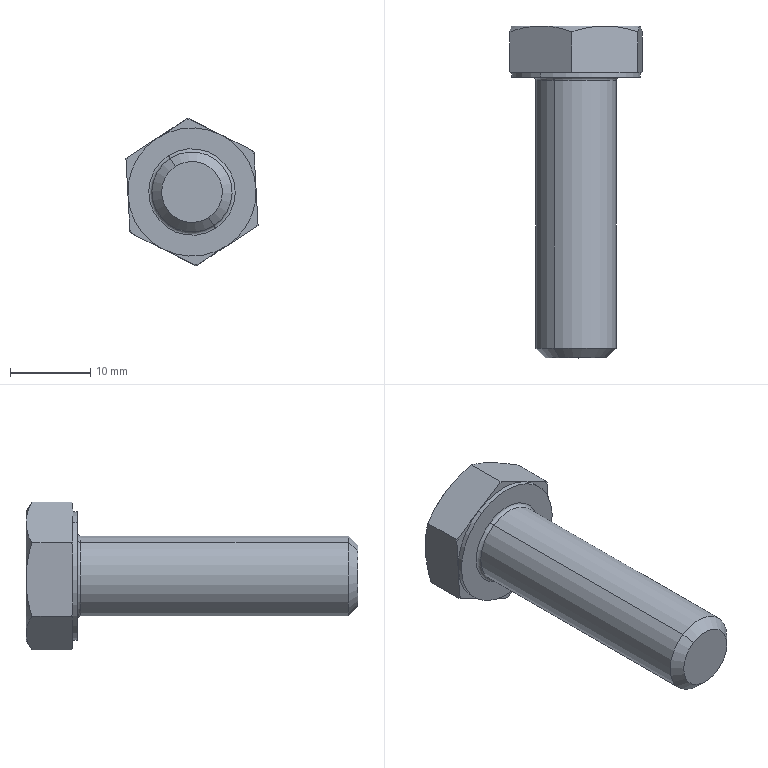Component | SolidWorks | 14HexHeadBolt_GradeAAndB[GBT5782-2000][M10_35_35]-1 | 1 solid | 35 faces | box 16.48 x 41.4 x 18.45 mm | volume 4131 mm3 | plane 15 | cone 14 | cylinder 4 | torus 2 | commonest cylinder face diameters 10 x2 16 x2 | material Steel
STEP:
#1=COLOUR_RGB('',0.7922,0.8196,0.9333);
#2=FILL_AREA_STYLE_COLOUR('',#1);
#3=FILL_AREA_STYLE('',(#2));
#4=SURFACE_STYLE_FILL_AREA(#3);
#5=SURFACE_SIDE_STYLE('',(#4));
#6=SURFACE_STYLE_USAGE(.BOTH.,#5);
#7=PRESENTATION_STYLE_ASSIGNMENT((#6));
#8=CARTESIAN_POINT('',(-7.986,6.04,16.976));
#9=VERTEX_POINT('',#8);
#10=CARTESIAN_POINT('',(-7.771,6.04,16.646));
#11=VERTEX_POINT('',#10);
#12=CARTESIAN_POINT('',(-7.879,6.04,16.811));
#13=DIRECTION('',(0.,-1.,0.));
#14=DIRECTION('',(0.5469,0.,-0.8372));
#15=AXIS2_PLACEMENT_3D('',#12,#13,#14);
#16=CIRCLE('',#15,0.1969);
#17=EDGE_CURVE('',#9,#11,#16,.T.);
#18=ORIENTED_EDGE('',*,*,#17,.F.);
#19=CARTESIAN_POINT('',(-7.995,6.055,16.989));
#20=VERTEX_POINT('',#19);
#21=CARTESIAN_POINT('',(-7.995,6.04,16.989));
#22=DIRECTION('',(0.8372,0.,0.5469));
#23=DIRECTION('',(0.5469,0.,-0.8372));
#24=AXIS2_PLACEMENT_3D('',#21,#22,#23);
#25=CIRCLE('',#24,0.01575);
#26=EDGE_CURVE('',#9,#20,#25,.T.);
#27=ORIENTED_EDGE('',*,*,#26,.T.);
#28=CARTESIAN_POINT('',(-7.762,6.055,16.633));
#29=VERTEX_POINT('',#28);
#30=CARTESIAN_POINT('',(-7.879,6.055,16.811));
#31=DIRECTION('',(0.,1.,0.));
#32=DIRECTION('',(0.5469,0.,-0.8372));
#33=AXIS2_PLACEMENT_3D('',#30,#31,#32);
#34=CIRCLE('',#33,0.2126);
#35=EDGE_CURVE('',#29,#20,#34,.T.);
#36=ORIENTED_EDGE('',*,*,#35,.F.);
#37=CARTESIAN_POINT('',(-7.762,6.04,16.633));
#38=DIRECTION('',(-0.8372,0.,-0.5469));
#39=DIRECTION('',(-0.5469,0.,0.8372));
#40=AXIS2_PLACEMENT_3D('',#37,#38,#39);
#41=CIRCLE('',#40,0.01575);
#42=EDGE_CURVE('',#11,#29,#41,.T.);
#43=ORIENTED_EDGE('',*,*,#42,.F.);
#44=EDGE_LOOP('',(#18,#27,#36,#43));
#45=FACE_OUTER_BOUND('',#44,.T.);
#46=CARTESIAN_POINT('',(-7.879,6.04,16.811));
#47=DIRECTION('',(0.,-1.,0.));
#48=DIRECTION('',(0.5469,0.,-0.8372));
#49=AXIS2_PLACEMENT_3D('',#46,#47,#48);
#50=TOROIDAL_SURFACE('',#49,0.2126,0.01575);
#51=ADVANCED_FACE('',(#45),#50,.F.);
#52=CARTESIAN_POINT('',(-7.797,4.678,16.686));
#53=VERTEX_POINT('',#52);
#54=CARTESIAN_POINT('',(-7.96,4.678,16.936));
#55=VERTEX_POINT('',#54);
#56=CARTESIAN_POINT('',(-7.879,4.678,16.811));
#57=DIRECTION('',(0.,-1.,0.));
#58=DIRECTION('',(-0.5469,0.,0.8372));
#59=AXIS2_PLACEMENT_3D('',#56,#57,#58);
#60=CIRCLE('',#59,0.1496);
#61=EDGE_CURVE('',#53,#55,#60,.T.);
#62=ORIENTED_EDGE('',*,*,#61,.F.);
#63=CARTESIAN_POINT('',(-7.771,4.725,16.646));
#64=VERTEX_POINT('',#63);
#65=CARTESIAN_POINT('',(-7.771,4.725,16.646));
#66=DIRECTION('',(0.3867,0.7071,-0.592));
#67=VECTOR('',#66,39.37);
#68=LINE('',#65,#67);
#69=EDGE_CURVE('',#53,#64,#68,.T.);
#70=ORIENTED_EDGE('',*,*,#69,.T.);
#71=CARTESIAN_POINT('',(-7.986,4.725,16.976));
#72=VERTEX_POINT('',#71);
#73=CARTESIAN_POINT('',(-7.879,4.725,16.811));
#74=DIRECTION('',(0.,1.,0.));
#75=DIRECTION('',(-0.5469,0.,0.8372));
#76=AXIS2_PLACEMENT_3D('',#73,#74,#75);
#77=CIRCLE('',#76,0.1969);
#78=EDGE_CURVE('',#72,#64,#77,.T.);
#79=ORIENTED_EDGE('',*,*,#78,.F.);
#80=CARTESIAN_POINT('',(-7.986,4.725,16.976));
#81=DIRECTION('',(-0.3867,0.7071,0.592));
#82=VECTOR('',#81,39.37);
#83=LINE('',#80,#82);
#84=EDGE_CURVE('',#55,#72,#83,.T.);
#85=ORIENTED_EDGE('',*,*,#84,.F.);
#86=EDGE_LOOP('',(#62,#70,#79,#85));
#87=FACE_OUTER_BOUND('',#86,.T.);
#88=CARTESIAN_POINT('',(-7.879,4.725,16.811));
#89=DIRECTION('',(0.,1.,0.));
#90=DIRECTION('',(-0.5469,0.,0.8372));
#91=AXIS2_PLACEMENT_3D('',#88,#89,#90);
#92=CONICAL_SURFACE('',#91,0.1969,0.7854);
#93=ADVANCED_FACE('',(#87),#92,.T.);
#94=ORIENTED_EDGE('',*,*,#78,.T.);
#95=CARTESIAN_POINT('',(-7.771,6.307,16.646));
#96=DIRECTION('',(0.,1.,0.));
#97=VECTOR('',#96,39.37);
#98=LINE('',#95,#97);
#99=EDGE_CURVE('',#64,#11,#98,.T.);
#100=ORIENTED_EDGE('',*,*,#99,.T.);
#101=CARTESIAN_POINT('',(-7.879,6.04,16.811));
#102=DIRECTION('',(0.,-1.,0.));
#103=DIRECTION('',(0.5469,0.,-0.8372));
#104=AXIS2_PLACEMENT_3D('',#101,#102,#103);
#105=CIRCLE('',#104,0.1969);
#106=EDGE_CURVE('',#11,#9,#105,.T.);
#107=ORIENTED_EDGE('',*,*,#106,.T.);
#108=CARTESIAN_POINT('',(-7.986,6.307,16.976));
#109=DIRECTION('',(0.,1.,0.));
#110=VECTOR('',#109,39.37);
#111=LINE('',#108,#110);
#112=EDGE_CURVE('',#72,#9,#111,.T.);
#113=ORIENTED_EDGE('',*,*,#112,.F.);
#114=EDGE_LOOP('',(#94,#100,#107,#113));
#115=FACE_OUTER_BOUND('',#114,.T.);
#116=CARTESIAN_POINT('',(-7.879,6.307,16.811));
#117=DIRECTION('',(0.,1.,0.));
#118=DIRECTION('',(-0.5469,0.,0.8372));
#119=AXIS2_PLACEMENT_3D('',#116,#117,#118);
#120=CYLINDRICAL_SURFACE('',#119,0.1969);
#121=ADVANCED_FACE('',(#115),#120,.T.);
#122=CARTESIAN_POINT('',(-7.706,6.055,16.547));
#123=VERTEX_POINT('',#122);
#124=CARTESIAN_POINT('',(-8.051,6.055,17.075));
#125=VERTEX_POINT('',#124);
#126=CARTESIAN_POINT('',(-7.879,6.055,16.811));
#127=DIRECTION('',(0.,-1.,0.));
#128=DIRECTION('',(0.5469,0.,-0.8372));
#129=AXIS2_PLACEMENT_3D('',#126,#127,#128);
#130=CIRCLE('',#129,0.315);
#131=EDGE_CURVE('',#123,#125,#130,.T.);
#132=ORIENTED_EDGE('',*,*,#131,.F.);
#133=CARTESIAN_POINT('',(-7.706,6.079,16.547));
#134=VERTEX_POINT('',#133);
#135=CARTESIAN_POINT('',(-7.706,6.307,16.547));
#136=DIRECTION('',(0.,1.,0.));
#137=VECTOR('',#136,39.37);
#138=LINE('',#135,#137);
#139=EDGE_CURVE('',#123,#134,#138,.T.);
#140=ORIENTED_EDGE('',*,*,#139,.T.);
#141=CARTESIAN_POINT('',(-7.564,6.079,16.828));
#142=VERTEX_POINT('',#141);
#143=CARTESIAN_POINT('',(-7.879,6.079,16.811));
#144=DIRECTION('',(0.,1.,0.));
#145=DIRECTION('',(-0.5469,0.,0.8372));
#146=AXIS2_PLACEMENT_3D('',#143,#144,#145);
#147=CIRCLE('',#146,0.315);
#148=EDGE_CURVE('',#142,#134,#147,.T.);
#149=ORIENTED_EDGE('',*,*,#148,.F.);
#150=CARTESIAN_POINT('',(-7.736,6.079,17.092));
#151=VERTEX_POINT('',#150);
#152=CARTESIAN_POINT('',(-7.879,6.079,16.811));
#153=DIRECTION('',(0.,1.,0.));
#154=DIRECTION('',(-0.5469,0.,0.8372));
#155=AXIS2_PLACEMENT_3D('',#152,#153,#154);
#156=CIRCLE('',#155,0.315);
#157=EDGE_CURVE('',#151,#142,#156,.T.);
#158=ORIENTED_EDGE('',*,*,#157,.F.);
#159=CARTESIAN_POINT('',(-8.051,6.079,17.075));
#160=VERTEX_POINT('',#159);
#161=CARTESIAN_POINT('',(-7.879,6.079,16.811));
#162=DIRECTION('',(0.,1.,0.));
#163=DIRECTION('',(-0.5469,0.,0.8372));
#164=AXIS2_PLACEMENT_3D('',#161,#162,#163);
#165=CIRCLE('',#164,0.315);
#166=EDGE_CURVE('',#160,#151,#165,.T.);
#167=ORIENTED_EDGE('',*,*,#166,.F.);
#168=CARTESIAN_POINT('',(-8.051,6.307,17.075));
#169=DIRECTION('',(0.,1.,0.));
#170=VECTOR('',#169,39.37);
#171=LINE('',#168,#170);
#172=EDGE_CURVE('',#125,#160,#171,.T.);
#173=ORIENTED_EDGE('',*,*,#172,.F.);
#174=EDGE_LOOP('',(#132,#140,#149,#158,#167,#173));
#175=FACE_OUTER_BOUND('',#174,.T.);
#176=CARTESIAN_POINT('',(-7.879,6.307,16.811));
#177=DIRECTION('',(0.,1.,0.));
#178=DIRECTION('',(-0.5469,0.,0.8372));
#179=AXIS2_PLACEMENT_3D('',#176,#177,#178);
#180=CYLINDRICAL_SURFACE('',#179,0.315);
#181=ADVANCED_FACE('',(#175),#180,.T.);
#182=CARTESIAN_POINT('',(-7.555,6.079,16.663));
#183=VERTEX_POINT('',#182);
#184=CARTESIAN_POINT('',(-7.554,6.079,16.647));
#185=DIRECTION('',(-0.05508,0.,0.9985));
#186=VECTOR('',#185,39.37);
#187=LINE('',#184,#186);
#188=EDGE_CURVE('',#183,#142,#187,.T.);
#189=ORIENTED_EDGE('',*,*,#188,.F.);
#190=CARTESIAN_POINT('',(-7.554,6.084,16.647));
#191=VERTEX_POINT('',#190);
#192=CARTESIAN_POINT('',(-7.554,6.084,16.647));
#193=CARTESIAN_POINT('',(-7.554,6.082,16.652));
#194=CARTESIAN_POINT('',(-7.555,6.081,16.658));
#195=CARTESIAN_POINT('',(-7.555,6.079,16.663));
#196=B_SPLINE_CURVE_WITH_KNOTS('',3,(#192,#193,#194,#195),.UNSPECIFIED.,.F.,.F.,(4,4),(0.00000024,0.0004231),.UNSPECIFIED.);
#197=EDGE_CURVE('',#191,#183,#196,.T.);
#198=ORIENTED_EDGE('',*,*,#197,.F.);
#199=CARTESIAN_POINT('',(-7.554,6.279,16.647));
#200=VERTEX_POINT('',#199);
#201=CARTESIAN_POINT('',(-7.554,6.055,16.647));
#202=DIRECTION('',(0.,1.,0.));
#203=VECTOR('',#202,39.37);
#204=LINE('',#201,#203);
#205=EDGE_CURVE('',#191,#200,#204,.T.);
#206=ORIENTED_EDGE('',*,*,#205,.T.);
#207=CARTESIAN_POINT('',(-7.564,6.307,16.828));
#208=VERTEX_POINT('',#207);
#209=CARTESIAN_POINT('',(-7.564,6.307,16.828));
#210=CARTESIAN_POINT('',(-7.563,6.307,16.813));
#211=CARTESIAN_POINT('',(-7.562,6.307,16.797));
#212=CARTESIAN_POINT('',(-7.561,6.304,16.767));
#213=CARTESIAN_POINT('',(-7.56,6.302,16.752));
#214=CARTESIAN_POINT('',(-7.557,6.295,16.706));
#215=CARTESIAN_POINT('',(-7.556,6.288,16.676));
#216=CARTESIAN_POINT('',(-7.554,6.279,16.647));
#217=B_SPLINE_CURVE_WITH_KNOTS('',3,(#209,#210,#211,#212,#213,#214,#215,#216),.UNSPECIFIED.,.F.,.F.,(4,2,2,4),(0.004674,0.005838,0.007002,0.00933),.UNSPECIFIED.);
#218=EDGE_CURVE('',#208,#200,#217,.T.);
#219=ORIENTED_EDGE('',*,*,#218,.F.);
#220=CARTESIAN_POINT('',(-7.574,6.279,17.01));
#221=VERTEX_POINT('',#220);
#222=CARTESIAN_POINT('',(-7.574,6.279,17.01));
#223=CARTESIAN_POINT('',(-7.572,6.288,16.98));
#224=CARTESIAN_POINT('',(-7.571,6.295,16.95));
#225=CARTESIAN_POINT('',(-7.567,6.305,16.89));
#226=CARTESIAN_POINT('',(-7.566,6.307,16.859));
#227=CARTESIAN_POINT('',(-7.564,6.307,16.828));
#228=B_SPLINE_CURVE_WITH_KNOTS('',3,(#222,#223,#224,#225,#226,#227),.UNSPECIFIED.,.F.,.F.,(4,2,4),(0.00000024,0.002337,0.004674),.UNSPECIFIED.);
#229=EDGE_CURVE('',#221,#208,#228,.T.);
#230=ORIENTED_EDGE('',*,*,#229,.F.);
#231=CARTESIAN_POINT('',(-7.574,6.084,17.01));
#232=VERTEX_POINT('',#231);
#233=CARTESIAN_POINT('',(-7.574,6.055,17.01));
#234=DIRECTION('',(0.,1.,0.));
#235=VECTOR('',#234,39.37);
#236=LINE('',#233,#235);
#237=EDGE_CURVE('',#232,#221,#236,.T.);
#238=ORIENTED_EDGE('',*,*,#237,.F.);
#239=CARTESIAN_POINT('',(-7.573,6.079,16.994));
#240=VERTEX_POINT('',#239);
#241=CARTESIAN_POINT('',(-7.573,6.079,16.994));
#242=CARTESIAN_POINT('',(-7.573,6.081,16.999));
#243=CARTESIAN_POINT('',(-7.574,6.082,17.005));
#244=CARTESIAN_POINT('',(-7.574,6.084,17.01));
#245=B_SPLINE_CURVE_WITH_KNOTS('',3,(#241,#242,#243,#244),.UNSPECIFIED.,.F.,.F.,(4,4),(0.008907,0.00933),.UNSPECIFIED.);
#246=EDGE_CURVE('',#240,#232,#245,.T.);
#247=ORIENTED_EDGE('',*,*,#246,.F.);
#248=CARTESIAN_POINT('',(-7.554,6.079,16.647));
#249=DIRECTION('',(-0.05508,0.,0.9985));
#250=VECTOR('',#249,39.37);
#251=LINE('',#248,#250);
#252=EDGE_CURVE('',#142,#240,#251,.T.);
#253=ORIENTED_EDGE('',*,*,#252,.F.);
#254=EDGE_LOOP('',(#189,#198,#206,#219,#230,#238,#247,#253));
#255=FACE_OUTER_BOUND('',#254,.T.);
#256=CARTESIAN_POINT('',(-7.554,6.055,16.647));
#257=DIRECTION('',(-0.9985,0.,-0.05508));
#258=DIRECTION('',(0.05508,0.,-0.9985));
#259=AXIS2_PLACEMENT_3D('',#256,#257,#258);
#260=PLANE('',#259);
#261=ADVANCED_FACE('',(#255),#260,.F.);
#262=CARTESIAN_POINT('',(-7.589,6.079,17.017));
#263=VERTEX_POINT('',#262);
#264=CARTESIAN_POINT('',(-7.574,6.079,17.01));
#265=DIRECTION('',(-0.8923,0.,0.4515));
#266=VECTOR('',#265,39.37);
#267=LINE('',#264,#266);
#268=EDGE_CURVE('',#263,#151,#267,.T.);
#269=ORIENTED_EDGE('',*,*,#268,.F.);
#270=CARTESIAN_POINT('',(-7.574,6.084,17.01));
#271=CARTESIAN_POINT('',(-7.579,6.082,17.012));
#272=CARTESIAN_POINT('',(-7.584,6.081,17.015));
#273=CARTESIAN_POINT('',(-7.589,6.079,17.017));
#274=B_SPLINE_CURVE_WITH_KNOTS('',3,(#270,#271,#272,#273),.UNSPECIFIED.,.F.,.F.,(4,4),(0.00000024,0.0004231),.UNSPECIFIED.);
#275=EDGE_CURVE('',#232,#263,#274,.T.);
#276=ORIENTED_EDGE('',*,*,#275,.F.);
#277=ORIENTED_EDGE('',*,*,#237,.T.);
#278=CARTESIAN_POINT('',(-7.736,6.307,17.092));
#279=VERTEX_POINT('',#278);
#280=CARTESIAN_POINT('',(-7.736,6.307,17.092));
#281=CARTESIAN_POINT('',(-7.723,6.307,17.085));
#282=CARTESIAN_POINT('',(-7.709,6.307,17.078));
#283=CARTESIAN_POINT('',(-7.681,6.304,17.064));
#284=CARTESIAN_POINT('',(-7.668,6.302,17.057));
#285=CARTESIAN_POINT('',(-7.627,6.295,17.037));
#286=CARTESIAN_POINT('',(-7.601,6.288,17.023));
#287=CARTESIAN_POINT('',(-7.574,6.279,17.01));
#288=B_SPLINE_CURVE_WITH_KNOTS('',3,(#280,#281,#282,#283,#284,#285,#286,#287),.UNSPECIFIED.,.F.,.F.,(4,2,2,4),(0.004674,0.005838,0.007002,0.00933),.UNSPECIFIED.);
#289=EDGE_CURVE('',#279,#221,#288,.T.);
#290=ORIENTED_EDGE('',*,*,#289,.F.);
#291=CARTESIAN_POINT('',(-7.899,6.279,17.174));
#292=VERTEX_POINT('',#291);
#293=CARTESIAN_POINT('',(-7.899,6.279,17.174));
#294=CARTESIAN_POINT('',(-7.872,6.288,17.161));
#295=CARTESIAN_POINT('',(-7.845,6.295,17.147));
#296=CARTESIAN_POINT('',(-7.791,6.305,17.12));
#297=CARTESIAN_POINT('',(-7.764,6.307,17.106));
#298=CARTESIAN_POINT('',(-7.736,6.307,17.092));
#299=B_SPLINE_CURVE_WITH_KNOTS('',3,(#293,#294,#295,#296,#297,#298),.UNSPECIFIED.,.F.,.F.,(4,2,4),(0.00000024,0.002337,0.004674),.UNSPECIFIED.);
#300=EDGE_CURVE('',#292,#279,#299,.T.);
#301=ORIENTED_EDGE('',*,*,#300,.F.);
#302=CARTESIAN_POINT('',(-7.899,6.084,17.174));
#303=VERTEX_POINT('',#302);
#304=CARTESIAN_POINT('',(-7.899,6.055,17.174));
#305=DIRECTION('',(0.,1.,0.));
#306=VECTOR('',#305,39.37);
#307=LINE('',#304,#306);
#308=EDGE_CURVE('',#303,#292,#307,.T.);
#309=ORIENTED_EDGE('',*,*,#308,.F.);
#310=CARTESIAN_POINT('',(-7.884,6.079,17.167));
#311=VERTEX_POINT('',#310);
#312=CARTESIAN_POINT('',(-7.884,6.079,17.167));
#313=CARTESIAN_POINT('',(-7.889,6.081,17.169));
#314=CARTESIAN_POINT('',(-7.894,6.082,17.172));
#315=CARTESIAN_POINT('',(-7.899,6.084,17.174));
#316=B_SPLINE_CURVE_WITH_KNOTS('',3,(#312,#313,#314,#315),.UNSPECIFIED.,.F.,.F.,(4,4),(0.008907,0.00933),.UNSPECIFIED.);
#317=EDGE_CURVE('',#311,#303,#316,.T.);
#318=ORIENTED_EDGE('',*,*,#317,.F.);
#319=CARTESIAN_POINT('',(-7.574,6.079,17.01));
#320=DIRECTION('',(-0.8923,0.,0.4515));
#321=VECTOR('',#320,39.37);
#322=LINE('',#319,#321);
#323=EDGE_CURVE('',#151,#311,#322,.T.);
#324=ORIENTED_EDGE('',*,*,#323,.F.);
#325=EDGE_LOOP('',(#269,#276,#277,#290,#301,#309,#318,#324));
#326=FACE_OUTER_BOUND('',#325,.T.);
#327=CARTESIAN_POINT('',(-7.574,6.055,17.01));
#328=DIRECTION('',(-0.4515,0.,-0.8923));
#329=DIRECTION('',(0.8923,0.,-0.4515));
#330=AXIS2_PLACEMENT_3D('',#327,#328,#329);
#331=PLANE('',#330);
#332=ADVANCED_FACE('',(#326),#331,.F.);
#333=CARTESIAN_POINT('',(-7.912,6.079,17.165));
#334=VERTEX_POINT('',#333);
#335=CARTESIAN_POINT('',(-7.899,6.079,17.174));
#336=DIRECTION('',(-0.8372,0.,-0.5469));
#337=VECTOR('',#336,39.37);
#338=LINE('',#335,#337);
#339=EDGE_CURVE('',#334,#160,#338,.T.);
#340=ORIENTED_EDGE('',*,*,#339,.F.);
#341=CARTESIAN_POINT('',(-7.899,6.084,17.174));
#342=CARTESIAN_POINT('',(-7.903,6.082,17.171));
#343=CARTESIAN_POINT('',(-7.908,6.081,17.168));
#344=CARTESIAN_POINT('',(-7.912,6.079,17.165));
#345=B_SPLINE_CURVE_WITH_KNOTS('',3,(#341,#342,#343,#344),.UNSPECIFIED.,.F.,.F.,(4,4),(0.02285,0.02328),.UNSPECIFIED.);
#346=EDGE_CURVE('',#303,#334,#345,.T.);
#347=ORIENTED_EDGE('',*,*,#346,.F.);
#348=ORIENTED_EDGE('',*,*,#308,.T.);
#349=CARTESIAN_POINT('',(-8.051,6.307,17.075));
#350=VERTEX_POINT('',#349);
#351=CARTESIAN_POINT('',(-8.051,6.307,17.075));
#352=CARTESIAN_POINT('',(-8.038,6.307,17.083));
#353=CARTESIAN_POINT('',(-8.025,6.307,17.092));
#354=CARTESIAN_POINT('',(-7.999,6.304,17.109));
#355=CARTESIAN_POINT('',(-7.986,6.302,17.117));
#356=CARTESIAN_POINT('',(-7.948,6.295,17.142));
#357=CARTESIAN_POINT('',(-7.923,6.288,17.158));
#358=CARTESIAN_POINT('',(-7.899,6.279,17.174));
#359=B_SPLINE_CURVE_WITH_KNOTS('',3,(#351,#352,#353,#354,#355,#356,#357,#358),.UNSPECIFIED.,.F.,.F.,(4,2,2,4),(0.01337,0.01454,0.01571,0.01805),.UNSPECIFIED.);
#360=EDGE_CURVE('',#350,#292,#359,.T.);
#361=ORIENTED_EDGE('',*,*,#360,.F.);
#362=CARTESIAN_POINT('',(-8.203,6.279,16.975));
#363=VERTEX_POINT('',#362);
#364=CARTESIAN_POINT('',(-8.203,6.279,16.975));
#365=CARTESIAN_POINT('',(-8.178,6.288,16.991));
#366=CARTESIAN_POINT('',(-8.153,6.295,17.008));
#367=CARTESIAN_POINT('',(-8.102,6.305,17.041));
#368=CARTESIAN_POINT('',(-8.077,6.307,17.058));
#369=CARTESIAN_POINT('',(-8.051,6.307,17.075));
#370=B_SPLINE_CURVE_WITH_KNOTS('',3,(#364,#365,#366,#367,#368,#369),.UNSPECIFIED.,.F.,.F.,(4,2,4),(0.00869,0.01103,0.01337),.UNSPECIFIED.);
#371=EDGE_CURVE('',#363,#350,#370,.T.);
#372=ORIENTED_EDGE('',*,*,#371,.F.);
#373=CARTESIAN_POINT('',(-8.203,6.084,16.975));
#374=VERTEX_POINT('',#373);
#375=CARTESIAN_POINT('',(-8.203,6.055,16.975));
#376=DIRECTION('',(0.,1.,0.));
#377=VECTOR('',#376,39.37);
#378=LINE('',#375,#377);
#379=EDGE_CURVE('',#374,#363,#378,.T.);
#380=ORIENTED_EDGE('',*,*,#379,.F.);
#381=CARTESIAN_POINT('',(-8.19,6.079,16.984));
#382=VERTEX_POINT('',#381);
#383=CARTESIAN_POINT('',(-8.19,6.079,16.984));
#384=CARTESIAN_POINT('',(-8.194,6.081,16.981));
#385=CARTESIAN_POINT('',(-8.199,6.082,16.978));
#386=CARTESIAN_POINT('',(-8.203,6.084,16.975));
#387=B_SPLINE_CURVE_WITH_KNOTS('',3,(#383,#384,#385,#386),.UNSPECIFIED.,.F.,.F.,(4,4),(0.03178,0.03221),.UNSPECIFIED.);
#388=EDGE_CURVE('',#382,#374,#387,.T.);
#389=ORIENTED_EDGE('',*,*,#388,.F.);
#390=CARTESIAN_POINT('',(-7.899,6.079,17.174));
#391=DIRECTION('',(-0.8372,0.,-0.5469));
#392=VECTOR('',#391,39.37);
#393=LINE('',#390,#392);
#394=EDGE_CURVE('',#160,#382,#393,.T.);
#395=ORIENTED_EDGE('',*,*,#394,.F.);
#396=EDGE_LOOP('',(#340,#347,#348,#361,#372,#380,#389,#395));
#397=FACE_OUTER_BOUND('',#396,.T.);
#398=CARTESIAN_POINT('',(-7.899,6.055,17.174));
#399=DIRECTION('',(0.5469,0.,-0.8372));
#400=DIRECTION('',(0.,1.,0.));
#401=AXIS2_PLACEMENT_3D('',#398,#399,#400);
#402=PLANE('',#401);
#403=ADVANCED_FACE('',(#397),#402,.F.);
#404=CARTESIAN_POINT('',(-8.202,6.079,16.959));
#405=VERTEX_POINT('',#404);
#406=CARTESIAN_POINT('',(-8.193,6.079,16.794));
#407=VERTEX_POINT('',#406);
#408=CARTESIAN_POINT('',(-8.183,6.079,16.612));
#409=DIRECTION('',(0.05508,0.,-0.9985));
#410=VECTOR('',#409,39.37);
#411=LINE('',#408,#410);
#412=EDGE_CURVE('',#405,#407,#411,.T.);
#413=ORIENTED_EDGE('',*,*,#412,.F.);
#414=CARTESIAN_POINT('',(-8.203,6.084,16.975));
#415=CARTESIAN_POINT('',(-8.203,6.082,16.97));
#416=CARTESIAN_POINT('',(-8.202,6.081,16.964));
#417=CARTESIAN_POINT('',(-8.202,6.079,16.959));
#418=B_SPLINE_CURVE_WITH_KNOTS('',3,(#414,#415,#416,#417),.UNSPECIFIED.,.F.,.F.,(4,4),(0.00000024,0.0004231),.UNSPECIFIED.);
#419=EDGE_CURVE('',#374,#405,#418,.T.);
#420=ORIENTED_EDGE('',*,*,#419,.F.);
#421=ORIENTED_EDGE('',*,*,#379,.T.);
#422=CARTESIAN_POINT('',(-8.193,6.307,16.794));
#423=VERTEX_POINT('',#422);
#424=CARTESIAN_POINT('',(-8.193,6.307,16.794));
#425=CARTESIAN_POINT('',(-8.194,6.307,16.809));
#426=CARTESIAN_POINT('',(-8.195,6.307,16.825));
#427=CARTESIAN_POINT('',(-8.196,6.304,16.855));
#428=CARTESIAN_POINT('',(-8.197,6.302,16.87));
#429=CARTESIAN_POINT('',(-8.2,6.295,16.916));
#430=CARTESIAN_POINT('',(-8.201,6.288,16.946));
#431=CARTESIAN_POINT('',(-8.203,6.279,16.975));
#432=B_SPLINE_CURVE_WITH_KNOTS('',3,(#424,#425,#426,#427,#428,#429,#430,#431),.UNSPECIFIED.,.F.,.F.,(4,2,2,4),(0.004674,0.005838,0.007002,0.00933),.UNSPECIFIED.);
#433=EDGE_CURVE('',#423,#363,#432,.T.);
#434=ORIENTED_EDGE('',*,*,#433,.F.);
#435=CARTESIAN_POINT('',(-8.183,6.279,16.612));
#436=VERTEX_POINT('',#435);
#437=CARTESIAN_POINT('',(-8.183,6.279,16.612));
#438=CARTESIAN_POINT('',(-8.185,6.288,16.642));
#439=CARTESIAN_POINT('',(-8.186,6.295,16.672));
#440=CARTESIAN_POINT('',(-8.19,6.305,16.732));
#441=CARTESIAN_POINT('',(-8.191,6.307,16.763));
#442=CARTESIAN_POINT('',(-8.193,6.307,16.794));
#443=B_SPLINE_CURVE_WITH_KNOTS('',3,(#437,#438,#439,#440,#441,#442),.UNSPECIFIED.,.F.,.F.,(4,2,4),(0.00000024,0.002337,0.004674),.UNSPECIFIED.);
#444=EDGE_CURVE('',#436,#423,#443,.T.);
#445=ORIENTED_EDGE('',*,*,#444,.F.);
#446=CARTESIAN_POINT('',(-8.183,6.084,16.612));
#447=VERTEX_POINT('',#446);
#448=CARTESIAN_POINT('',(-8.183,6.055,16.612));
#449=DIRECTION('',(0.,1.,0.));
#450=VECTOR('',#449,39.37);
#451=LINE('',#448,#450);
#452=EDGE_CURVE('',#447,#436,#451,.T.);
#453=ORIENTED_EDGE('',*,*,#452,.F.);
#454=CARTESIAN_POINT('',(-8.184,6.079,16.628));
#455=VERTEX_POINT('',#454);
#456=CARTESIAN_POINT('',(-8.184,6.079,16.628));
#457=CARTESIAN_POINT('',(-8.184,6.081,16.623));
#458=CARTESIAN_POINT('',(-8.183,6.082,16.617));
#459=CARTESIAN_POINT('',(-8.183,6.084,16.612));
#460=B_SPLINE_CURVE_WITH_KNOTS('',3,(#456,#457,#458,#459),.UNSPECIFIED.,.F.,.F.,(4,4),(0.008907,0.00933),.UNSPECIFIED.);
#461=EDGE_CURVE('',#455,#447,#460,.T.);
#462=ORIENTED_EDGE('',*,*,#461,.F.);
#463=CARTESIAN_POINT('',(-8.183,6.079,16.612));
#464=DIRECTION('',(0.05508,0.,-0.9985));
#465=VECTOR('',#464,39.37);
#466=LINE('',#463,#465);
#467=EDGE_CURVE('',#407,#455,#466,.T.);
#468=ORIENTED_EDGE('',*,*,#467,.F.);
#469=EDGE_LOOP('',(#413,#420,#421,#434,#445,#453,#462,#468));
#470=FACE_OUTER_BOUND('',#469,.T.);
#471=CARTESIAN_POINT('',(-8.183,6.055,16.612));
#472=DIRECTION('',(0.9985,0.,0.05508));
#473=DIRECTION('',(-0.05508,0.,0.9985));
#474=AXIS2_PLACEMENT_3D('',#471,#472,#473);
#475=PLANE('',#474);
#476=ADVANCED_FACE('',(#470),#475,.F.);
#477=CARTESIAN_POINT('',(-8.169,6.079,16.605));
#478=VERTEX_POINT('',#477);
#479=CARTESIAN_POINT('',(-8.021,6.079,16.53));
#480=VERTEX_POINT('',#479);
#481=CARTESIAN_POINT('',(-7.859,6.079,16.448));
#482=DIRECTION('',(0.8923,0.,-0.4515));
#483=VECTOR('',#482,39.37);
#484=LINE('',#481,#483);
#485=EDGE_CURVE('',#478,#480,#484,.T.);
#486=ORIENTED_EDGE('',*,*,#485,.F.);
#487=CARTESIAN_POINT('',(-8.183,6.084,16.612));
#488=CARTESIAN_POINT('',(-8.178,6.082,16.61));
#489=CARTESIAN_POINT('',(-8.173,6.081,16.607));
#490=CARTESIAN_POINT('',(-8.169,6.079,16.605));
#491=B_SPLINE_CURVE_WITH_KNOTS('',3,(#487,#488,#489,#490),.UNSPECIFIED.,.F.,.F.,(4,4),(0.00000024,0.0004231),.UNSPECIFIED.);
#492=EDGE_CURVE('',#447,#478,#491,.T.);
#493=ORIENTED_EDGE('',*,*,#492,.F.);
#494=ORIENTED_EDGE('',*,*,#452,.T.);
#495=CARTESIAN_POINT('',(-8.021,6.307,16.53));
#496=VERTEX_POINT('',#495);
#497=CARTESIAN_POINT('',(-8.021,6.307,16.53));
#498=CARTESIAN_POINT('',(-8.035,6.307,16.537));
#499=CARTESIAN_POINT('',(-8.048,6.307,16.544));
#500=CARTESIAN_POINT('',(-8.076,6.304,16.558));
#501=CARTESIAN_POINT('',(-8.089,6.302,16.565));
#502=CARTESIAN_POINT('',(-8.13,6.295,16.585));
#503=CARTESIAN_POINT('',(-8.157,6.288,16.599));
#504=CARTESIAN_POINT('',(-8.183,6.279,16.612));
#505=B_SPLINE_CURVE_WITH_KNOTS('',3,(#497,#498,#499,#500,#501,#502,#503,#504),.UNSPECIFIED.,.F.,.F.,(4,2,2,4),(0.004674,0.005838,0.007002,0.00933),.UNSPECIFIED.);
#506=EDGE_CURVE('',#496,#436,#505,.T.);
#507=ORIENTED_EDGE('',*,*,#506,.F.);
#508=CARTESIAN_POINT('',(-7.859,6.279,16.448));
#509=VERTEX_POINT('',#508);
#510=CARTESIAN_POINT('',(-7.859,6.279,16.448));
#511=CARTESIAN_POINT('',(-7.885,6.288,16.461));
#512=CARTESIAN_POINT('',(-7.912,6.295,16.475));
#513=CARTESIAN_POINT('',(-7.966,6.305,16.502));
#514=CARTESIAN_POINT('',(-7.993,6.307,16.516));
#515=CARTESIAN_POINT('',(-8.021,6.307,16.53));
#516=B_SPLINE_CURVE_WITH_KNOTS('',3,(#510,#511,#512,#513,#514,#515),.UNSPECIFIED.,.F.,.F.,(4,2,4),(0.00000024,0.002337,0.004674),.UNSPECIFIED.);
#517=EDGE_CURVE('',#509,#496,#516,.T.);
#518=ORIENTED_EDGE('',*,*,#517,.F.);
#519=CARTESIAN_POINT('',(-7.859,6.084,16.448));
#520=VERTEX_POINT('',#519);
#521=CARTESIAN_POINT('',(-7.859,6.055,16.448));
#522=DIRECTION('',(0.,1.,0.));
#523=VECTOR('',#522,39.37);
#524=LINE('',#521,#523);
#525=EDGE_CURVE('',#520,#509,#524,.T.);
#526=ORIENTED_EDGE('',*,*,#525,.F.);
#527=CARTESIAN_POINT('',(-7.873,6.079,16.455));
#528=VERTEX_POINT('',#527);
#529=CARTESIAN_POINT('',(-7.873,6.079,16.455));
#530=CARTESIAN_POINT('',(-7.868,6.081,16.453));
#531=CARTESIAN_POINT('',(-7.863,6.082,16.45));
#532=CARTESIAN_POINT('',(-7.859,6.084,16.448));
#533=B_SPLINE_CURVE_WITH_KNOTS('',3,(#529,#530,#531,#532),.UNSPECIFIED.,.F.,.F.,(4,4),(0.008907,0.00933),.UNSPECIFIED.);
#534=EDGE_CURVE('',#528,#520,#533,.T.);
#535=ORIENTED_EDGE('',*,*,#534,.F.);
#536=CARTESIAN_POINT('',(-7.859,6.079,16.448));
#537=DIRECTION('',(0.8923,0.,-0.4515));
#538=VECTOR('',#537,39.37);
#539=LINE('',#536,#538);
#540=EDGE_CURVE('',#480,#528,#539,.T.);
#541=ORIENTED_EDGE('',*,*,#540,.F.);
#542=EDGE_LOOP('',(#486,#493,#494,#507,#518,#526,#535,#541));
#543=FACE_OUTER_BOUND('',#542,.T.);
#544=CARTESIAN_POINT('',(-7.859,6.055,16.448));
#545=DIRECTION('',(0.4515,0.,0.8923));
#546=DIRECTION('',(-0.8923,0.,0.4515));
#547=AXIS2_PLACEMENT_3D('',#544,#545,#546);
#548=PLANE('',#547);
#549=ADVANCED_FACE('',(#543),#548,.F.);
#550=CARTESIAN_POINT('',(-7.845,6.079,16.457));
#551=VERTEX_POINT('',#550);
#552=CARTESIAN_POINT('',(-7.554,6.079,16.647));
#553=DIRECTION('',(0.8372,0.,0.5469));
#554=VECTOR('',#553,39.37);
#555=LINE('',#552,#554);
#556=EDGE_CURVE('',#551,#134,#555,.T.);
#557=ORIENTED_EDGE('',*,*,#556,.F.);
#558=CARTESIAN_POINT('',(-7.859,6.084,16.448));
#559=CARTESIAN_POINT('',(-7.854,6.082,16.451));
#560=CARTESIAN_POINT('',(-7.85,6.081,16.454));
#561=CARTESIAN_POINT('',(-7.845,6.079,16.457));
#562=B_SPLINE_CURVE_WITH_KNOTS('',3,(#558,#559,#560,#561),.UNSPECIFIED.,.F.,.F.,(4,4),(0.00869,0.009114),.UNSPECIFIED.);
#563=EDGE_CURVE('',#520,#551,#562,.T.);
#564=ORIENTED_EDGE('',*,*,#563,.F.);
#565=ORIENTED_EDGE('',*,*,#525,.T.);
#566=CARTESIAN_POINT('',(-7.706,6.307,16.547));
#567=VERTEX_POINT('',#566);
#568=CARTESIAN_POINT('',(-7.706,6.307,16.547));
#569=CARTESIAN_POINT('',(-7.732,6.307,16.531));
#570=CARTESIAN_POINT('',(-7.758,6.305,16.514));
#571=CARTESIAN_POINT('',(-7.808,6.295,16.481));
#572=CARTESIAN_POINT('',(-7.834,6.288,16.464));
#573=CARTESIAN_POINT('',(-7.859,6.279,16.448));
#574=B_SPLINE_CURVE_WITH_KNOTS('',3,(#568,#569,#570,#571,#572,#573),.UNSPECIFIED.,.F.,.F.,(4,2,4),(0.02753,0.02987,0.03221),.UNSPECIFIED.);
#575=EDGE_CURVE('',#567,#509,#574,.T.);
#576=ORIENTED_EDGE('',*,*,#575,.F.);
#577=CARTESIAN_POINT('',(-7.554,6.279,16.647));
#578=CARTESIAN_POINT('',(-7.579,6.288,16.631));
#579=CARTESIAN_POINT('',(-7.604,6.295,16.614));
#580=CARTESIAN_POINT('',(-7.642,6.302,16.59));
#581=CARTESIAN_POINT('',(-7.655,6.304,16.581));
#582=CARTESIAN_POINT('',(-7.68,6.307,16.564));
#583=CARTESIAN_POINT('',(-7.693,6.307,16.556));
#584=CARTESIAN_POINT('',(-7.706,6.307,16.547));
#585=B_SPLINE_CURVE_WITH_KNOTS('',3,(#577,#578,#579,#580,#581,#582,#583,#584),.UNSPECIFIED.,.F.,.F.,(4,2,2,4),(0.02285,0.02519,0.02636,0.02753),.UNSPECIFIED.);
#586=EDGE_CURVE('',#200,#567,#585,.T.);
#587=ORIENTED_EDGE('',*,*,#586,.F.);
#588=ORIENTED_EDGE('',*,*,#205,.F.);
#589=CARTESIAN_POINT('',(-7.568,6.079,16.638));
#590=VERTEX_POINT('',#589);
#591=CARTESIAN_POINT('',(-7.568,6.079,16.638));
#592=CARTESIAN_POINT('',(-7.563,6.081,16.641));
#593=CARTESIAN_POINT('',(-7.559,6.082,16.644));
#594=CARTESIAN_POINT('',(-7.554,6.084,16.647));
#595=B_SPLINE_CURVE_WITH_KNOTS('',3,(#591,#592,#593,#594),.UNSPECIFIED.,.F.,.F.,(4,4),(0.01762,0.01805),.UNSPECIFIED.);
#596=EDGE_CURVE('',#590,#191,#595,.T.);
#597=ORIENTED_EDGE('',*,*,#596,.F.);
#598=CARTESIAN_POINT('',(-7.554,6.079,16.647));
#599=DIRECTION('',(0.8372,0.,0.5469));
#600=VECTOR('',#599,39.37);
#601=LINE('',#598,#600);
#602=EDGE_CURVE('',#134,#590,#601,.T.);
#603=ORIENTED_EDGE('',*,*,#602,.F.);
#604=EDGE_LOOP('',(#557,#564,#565,#576,#587,#588,#597,#603));
#605=FACE_OUTER_BOUND('',#604,.T.);
#606=CARTESIAN_POINT('',(-7.554,6.055,16.647));
#607=DIRECTION('',(-0.5469,0.,0.8372));
#608=DIRECTION('',(-0.8372,0.,-0.5469));
#609=AXIS2_PLACEMENT_3D('',#606,#607,#608);
#610=PLANE('',#609);
#611=ADVANCED_FACE('',(#605),#610,.F.);
#612=ORIENTED_EDGE('',*,*,#563,.T.);
#613=CARTESIAN_POINT('',(-7.879,6.079,16.811));
#614=DIRECTION('',(0.,1.,0.));
#615=DIRECTION('',(0.5469,0.,-0.8372));
#616=AXIS2_PLACEMENT_3D('',#613,#614,#615);
#617=CIRCLE('',#616,0.3559);
#618=EDGE_CURVE('',#551,#528,#617,.T.);
#619=ORIENTED_EDGE('',*,*,#618,.T.);
#620=ORIENTED_EDGE('',*,*,#534,.T.);
#621=EDGE_LOOP('',(#612,#619,#620));
#622=FACE_OUTER_BOUND('',#621,.T.);
#623=CARTESIAN_POINT('',(-7.879,6.197,16.811));
#624=DIRECTION('',(0.,1.,0.));
#625=DIRECTION('',(-0.5469,0.,0.8372));
#626=AXIS2_PLACEMENT_3D('',#623,#624,#625);
#627=CONICAL_SURFACE('',#626,0.5605,1.047);
#628=ADVANCED_FACE('',(#622),#627,.T.);
#629=ORIENTED_EDGE('',*,*,#492,.T.);
#630=CARTESIAN_POINT('',(-7.879,6.079,16.811));
#631=DIRECTION('',(0.,1.,0.));
#632=DIRECTION('',(0.5469,0.,-0.8372));
#633=AXIS2_PLACEMENT_3D('',#630,#631,#632);
#634=CIRCLE('',#633,0.3559);
#635=EDGE_CURVE('',#478,#455,#634,.T.);
#636=ORIENTED_EDGE('',*,*,#635,.T.);
#637=ORIENTED_EDGE('',*,*,#461,.T.);
#638=EDGE_LOOP('',(#629,#636,#637));
#639=FACE_OUTER_BOUND('',#638,.T.);
#640=CARTESIAN_POINT('',(-7.879,6.197,16.811));
#641=DIRECTION('',(0.,1.,0.));
#642=DIRECTION('',(-0.5469,0.,0.8372));
#643=AXIS2_PLACEMENT_3D('',#640,#641,#642);
#644=CONICAL_SURFACE('',#643,0.5605,1.047);
#645=ADVANCED_FACE('',(#639),#644,.T.);
#646=ORIENTED_EDGE('',*,*,#419,.T.);
#647=CARTESIAN_POINT('',(-7.879,6.079,16.811));
#648=DIRECTION('',(0.,1.,0.));
#649=DIRECTION('',(0.5469,0.,-0.8372));
#650=AXIS2_PLACEMENT_3D('',#647,#648,#649);
#651=CIRCLE('',#650,0.3559);
#652=EDGE_CURVE('',#405,#382,#651,.T.);
#653=ORIENTED_EDGE('',*,*,#652,.T.);
#654=ORIENTED_EDGE('',*,*,#388,.T.);
#655=EDGE_LOOP('',(#646,#653,#654));
#656=FACE_OUTER_BOUND('',#655,.T.);
#657=CARTESIAN_POINT('',(-7.879,6.197,16.811));
#658=DIRECTION('',(0.,1.,0.));
#659=DIRECTION('',(-0.5469,0.,0.8372));
#660=AXIS2_PLACEMENT_3D('',#657,#658,#659);
#661=CONICAL_SURFACE('',#660,0.5605,1.047);
#662=ADVANCED_FACE('',(#656),#661,.T.);
#663=ORIENTED_EDGE('',*,*,#346,.T.);
#664=CARTESIAN_POINT('',(-7.879,6.079,16.811));
#665=DIRECTION('',(0.,1.,0.));
#666=DIRECTION('',(0.5469,0.,-0.8372));
#667=AXIS2_PLACEMENT_3D('',#664,#665,#666);
#668=CIRCLE('',#667,0.3559);
#669=EDGE_CURVE('',#334,#311,#668,.T.);
#670=ORIENTED_EDGE('',*,*,#669,.T.);
#671=ORIENTED_EDGE('',*,*,#317,.T.);
#672=EDGE_LOOP('',(#663,#670,#671));
#673=FACE_OUTER_BOUND('',#672,.T.);
#674=CARTESIAN_POINT('',(-7.879,6.197,16.811));
#675=DIRECTION('',(0.,1.,0.));
#676=DIRECTION('',(-0.5469,0.,0.8372));
#677=AXIS2_PLACEMENT_3D('',#674,#675,#676);
#678=CONICAL_SURFACE('',#677,0.5605,1.047);
#679=ADVANCED_FACE('',(#673),#678,.T.);
#680=ORIENTED_EDGE('',*,*,#275,.T.);
#681=CARTESIAN_POINT('',(-7.879,6.079,16.811));
#682=DIRECTION('',(0.,1.,0.));
#683=DIRECTION('',(0.5469,0.,-0.8372));
#684=AXIS2_PLACEMENT_3D('',#681,#682,#683);
#685=CIRCLE('',#684,0.3559);
#686=EDGE_CURVE('',#263,#240,#685,.T.);
#687=ORIENTED_EDGE('',*,*,#686,.T.);
#688=ORIENTED_EDGE('',*,*,#246,.T.);
#689=EDGE_LOOP('',(#680,#687,#688));
#690=FACE_OUTER_BOUND('',#689,.T.);
#691=CARTESIAN_POINT('',(-7.879,6.197,16.811));
#692=DIRECTION('',(0.,1.,0.));
#693=DIRECTION('',(-0.5469,0.,0.8372));
#694=AXIS2_PLACEMENT_3D('',#691,#692,#693);
#695=CONICAL_SURFACE('',#694,0.5605,1.047);
#696=ADVANCED_FACE('',(#690),#695,.T.);
#697=ORIENTED_EDGE('',*,*,#197,.T.);
#698=CARTESIAN_POINT('',(-7.879,6.079,16.811));
#699=DIRECTION('',(0.,1.,0.));
#700=DIRECTION('',(0.5469,0.,-0.8372));
#701=AXIS2_PLACEMENT_3D('',#698,#699,#700);
#702=CIRCLE('',#701,0.3559);
#703=EDGE_CURVE('',#183,#590,#702,.T.);
#704=ORIENTED_EDGE('',*,*,#703,.T.);
#705=ORIENTED_EDGE('',*,*,#596,.T.);
#706=EDGE_LOOP('',(#697,#704,#705));
#707=FACE_OUTER_BOUND('',#706,.T.);
#708=CARTESIAN_POINT('',(-7.879,6.197,16.811));
#709=DIRECTION('',(0.,1.,0.));
#710=DIRECTION('',(-0.5469,0.,0.8372));
#711=AXIS2_PLACEMENT_3D('',#708,#709,#710);
#712=CONICAL_SURFACE('',#711,0.5605,1.047);
#713=ADVANCED_FACE('',(#707),#712,.T.);
#714=ORIENTED_EDGE('',*,*,#517,.T.);
#715=CARTESIAN_POINT('',(-7.879,6.307,16.811));
#716=DIRECTION('',(0.,-1.,0.));
#717=DIRECTION('',(0.5469,0.,-0.8372));
#718=AXIS2_PLACEMENT_3D('',#715,#716,#717);
#719=CIRCLE('',#718,0.315);
#720=EDGE_CURVE('',#496,#567,#719,.T.);
#721=ORIENTED_EDGE('',*,*,#720,.T.);
#722=ORIENTED_EDGE('',*,*,#575,.T.);
#723=EDGE_LOOP('',(#714,#721,#722));
#724=FACE_OUTER_BOUND('',#723,.T.);
#725=CARTESIAN_POINT('',(-7.879,6.307,16.811));
#726=DIRECTION('',(0.,-1.,0.));
#727=DIRECTION('',(0.5469,0.,-0.8372));
#728=AXIS2_PLACEMENT_3D('',#725,#726,#727);
#729=CONICAL_SURFACE('',#728,0.315,1.047);
#730=ADVANCED_FACE('',(#724),#729,.T.);
#731=ORIENTED_EDGE('',*,*,#444,.T.);
#732=CARTESIAN_POINT('',(-7.879,6.307,16.811));
#733=DIRECTION('',(0.,-1.,0.));
#734=DIRECTION('',(0.5469,0.,-0.8372));
#735=AXIS2_PLACEMENT_3D('',#732,#733,#734);
#736=CIRCLE('',#735,0.315);
#737=EDGE_CURVE('',#423,#496,#736,.T.);
#738=ORIENTED_EDGE('',*,*,#737,.T.);
#739=ORIENTED_EDGE('',*,*,#506,.T.);
#740=EDGE_LOOP('',(#731,#738,#739));
#741=FACE_OUTER_BOUND('',#740,.T.);
#742=CARTESIAN_POINT('',(-7.879,6.307,16.811));
#743=DIRECTION('',(0.,-1.,0.));
#744=DIRECTION('',(0.5469,0.,-0.8372));
#745=AXIS2_PLACEMENT_3D('',#742,#743,#744);
#746=CONICAL_SURFACE('',#745,0.315,1.047);
#747=ADVANCED_FACE('',(#741),#746,.T.);
#748=ORIENTED_EDGE('',*,*,#371,.T.);
#749=CARTESIAN_POINT('',(-7.879,6.307,16.811));
#750=DIRECTION('',(0.,-1.,0.));
#751=DIRECTION('',(0.5469,0.,-0.8372));
#752=AXIS2_PLACEMENT_3D('',#749,#750,#751);
#753=CIRCLE('',#752,0.315);
#754=EDGE_CURVE('',#350,#423,#753,.T.);
#755=ORIENTED_EDGE('',*,*,#754,.T.);
#756=ORIENTED_EDGE('',*,*,#433,.T.);
#757=EDGE_LOOP('',(#748,#755,#756));
#758=FACE_OUTER_BOUND('',#757,.T.);
#759=CARTESIAN_POINT('',(-7.879,6.307,16.811));
#760=DIRECTION('',(0.,-1.,0.));
#761=DIRECTION('',(0.5469,0.,-0.8372));
#762=AXIS2_PLACEMENT_3D('',#759,#760,#761);
#763=CONICAL_SURFACE('',#762,0.315,1.047);
#764=ADVANCED_FACE('',(#758),#763,.T.);
#765=ORIENTED_EDGE('',*,*,#360,.T.);
#766=ORIENTED_EDGE('',*,*,#300,.T.);
#767=CARTESIAN_POINT('',(-7.879,6.307,16.811));
#768=DIRECTION('',(0.,1.,0.));
#769=DIRECTION('',(-0.5469,0.,0.8372));
#770=AXIS2_PLACEMENT_3D('',#767,#768,#769);
#771=CIRCLE('',#770,0.315);
#772=EDGE_CURVE('',#350,#279,#771,.T.);
#773=ORIENTED_EDGE('',*,*,#772,.F.);
#774=EDGE_LOOP('',(#765,#766,#773));
#775=FACE_OUTER_BOUND('',#774,.T.);
#776=CARTESIAN_POINT('',(-7.879,6.307,16.811));
#777=DIRECTION('',(0.,-1.,0.));
#778=DIRECTION('',(0.5469,0.,-0.8372));
#779=AXIS2_PLACEMENT_3D('',#776,#777,#778);
#780=CONICAL_SURFACE('',#779,0.315,1.047);
#781=ADVANCED_FACE('',(#775),#780,.T.);
#782=ORIENTED_EDGE('',*,*,#289,.T.);
#783=ORIENTED_EDGE('',*,*,#229,.T.);
#784=CARTESIAN_POINT('',(-7.879,6.307,16.811));
#785=DIRECTION('',(0.,-1.,0.));
#786=DIRECTION('',(0.5469,0.,-0.8372));
#787=AXIS2_PLACEMENT_3D('',#784,#785,#786);
#788=CIRCLE('',#787,0.315);
#789=EDGE_CURVE('',#208,#279,#788,.T.);
#790=ORIENTED_EDGE('',*,*,#789,.T.);
#791=EDGE_LOOP('',(#782,#783,#790));
#792=FACE_OUTER_BOUND('',#791,.T.);
#793=CARTESIAN_POINT('',(-7.879,6.307,16.811));
#794=DIRECTION('',(0.,-1.,0.));
#795=DIRECTION('',(0.5469,0.,-0.8372));
#796=AXIS2_PLACEMENT_3D('',#793,#794,#795);
#797=CONICAL_SURFACE('',#796,0.315,1.047);
#798=ADVANCED_FACE('',(#792),#797,.T.);
#799=ORIENTED_EDGE('',*,*,#218,.T.);
#800=ORIENTED_EDGE('',*,*,#586,.T.);
#801=CARTESIAN_POINT('',(-7.879,6.307,16.811));
#802=DIRECTION('',(0.,-1.,0.));
#803=DIRECTION('',(0.5469,0.,-0.8372));
#804=AXIS2_PLACEMENT_3D('',#801,#802,#803);
#805=CIRCLE('',#804,0.315);
#806=EDGE_CURVE('',#567,#208,#805,.T.);
#807=ORIENTED_EDGE('',*,*,#806,.T.);
#808=EDGE_LOOP('',(#799,#800,#807));
#809=FACE_OUTER_BOUND('',#808,.T.);
#810=CARTESIAN_POINT('',(-7.879,6.307,16.811));
#811=DIRECTION('',(0.,-1.,0.));
#812=DIRECTION('',(0.5469,0.,-0.8372));
#813=AXIS2_PLACEMENT_3D('',#810,#811,#812);
#814=CONICAL_SURFACE('',#813,0.315,1.047);
#815=ADVANCED_FACE('',(#809),#814,.T.);
#816=ORIENTED_EDGE('',*,*,#806,.F.);
#817=ORIENTED_EDGE('',*,*,#720,.F.);
#818=ORIENTED_EDGE('',*,*,#737,.F.);
#819=ORIENTED_EDGE('',*,*,#754,.F.);
#820=ORIENTED_EDGE('',*,*,#772,.T.);
#821=ORIENTED_EDGE('',*,*,#789,.F.);
#822=EDGE_LOOP('',(#816,#817,#818,#819,#820,#821));
#823=FACE_OUTER_BOUND('',#822,.T.);
#824=CARTESIAN_POINT('',(-7.574,6.307,17.01));
#825=DIRECTION('',(0.,-1.,0.));
#826=DIRECTION('',(0.5469,0.,-0.8372));
#827=AXIS2_PLACEMENT_3D('',#824,#825,#826);
#828=PLANE('',#827);
#829=ADVANCED_FACE('',(#823),#828,.F.);
#830=ORIENTED_EDGE('',*,*,#394,.T.);
#831=ORIENTED_EDGE('',*,*,#652,.F.);
#832=ORIENTED_EDGE('',*,*,#412,.T.);
#833=CARTESIAN_POINT('',(-7.879,6.079,16.811));
#834=DIRECTION('',(0.,1.,0.));
#835=DIRECTION('',(-0.5469,0.,0.8372));
#836=AXIS2_PLACEMENT_3D('',#833,#834,#835);
#837=CIRCLE('',#836,0.315);
#838=EDGE_CURVE('',#407,#160,#837,.T.);
#839=ORIENTED_EDGE('',*,*,#838,.T.);
#840=EDGE_LOOP('',(#830,#831,#832,#839));
#841=FACE_OUTER_BOUND('',#840,.T.);
#842=CARTESIAN_POINT('',(-7.615,6.079,16.983));
#843=DIRECTION('',(0.,-1.,0.));
#844=DIRECTION('',(0.5469,0.,-0.8372));
#845=AXIS2_PLACEMENT_3D('',#842,#843,#844);
#846=PLANE('',#845);
#847=ADVANCED_FACE('',(#841),#846,.T.);
#848=ORIENTED_EDGE('',*,*,#268,.T.);
#849=ORIENTED_EDGE('',*,*,#157,.T.);
#850=ORIENTED_EDGE('',*,*,#252,.T.);
#851=ORIENTED_EDGE('',*,*,#686,.F.);
#852=EDGE_LOOP('',(#848,#849,#850,#851));
#853=FACE_OUTER_BOUND('',#852,.T.);
#854=CARTESIAN_POINT('',(-7.615,6.079,16.983));
#855=DIRECTION('',(0.,-1.,0.));
#856=DIRECTION('',(0.5469,0.,-0.8372));
#857=AXIS2_PLACEMENT_3D('',#854,#855,#856);
#858=PLANE('',#857);
#859=ADVANCED_FACE('',(#853),#858,.T.);
#860=ORIENTED_EDGE('',*,*,#467,.T.);
#861=ORIENTED_EDGE('',*,*,#635,.F.);
#862=ORIENTED_EDGE('',*,*,#485,.T.);
#863=CARTESIAN_POINT('',(-7.879,6.079,16.811));
#864=DIRECTION('',(0.,1.,0.));
#865=DIRECTION('',(-0.5469,0.,0.8372));
#866=AXIS2_PLACEMENT_3D('',#863,#864,#865);
#867=CIRCLE('',#866,0.315);
#868=EDGE_CURVE('',#480,#407,#867,.T.);
#869=ORIENTED_EDGE('',*,*,#868,.T.);
#870=EDGE_LOOP('',(#860,#861,#862,#869));
#871=FACE_OUTER_BOUND('',#870,.T.);
#872=CARTESIAN_POINT('',(-7.615,6.079,16.983));
#873=DIRECTION('',(0.,-1.,0.));
#874=DIRECTION('',(0.5469,0.,-0.8372));
#875=AXIS2_PLACEMENT_3D('',#872,#873,#874);
#876=PLANE('',#875);
#877=ADVANCED_FACE('',(#871),#876,.T.);
#878=ORIENTED_EDGE('',*,*,#540,.T.);
#879=ORIENTED_EDGE('',*,*,#618,.F.);
#880=ORIENTED_EDGE('',*,*,#556,.T.);
#881=CARTESIAN_POINT('',(-7.879,6.079,16.811));
#882=DIRECTION('',(0.,1.,0.));
#883=DIRECTION('',(-0.5469,0.,0.8372));
#884=AXIS2_PLACEMENT_3D('',#881,#882,#883);
#885=CIRCLE('',#884,0.315);
#886=EDGE_CURVE('',#134,#480,#885,.T.);
#887=ORIENTED_EDGE('',*,*,#886,.T.);
#888=EDGE_LOOP('',(#878,#879,#880,#887));
#889=FACE_OUTER_BOUND('',#888,.T.);
#890=CARTESIAN_POINT('',(-7.615,6.079,16.983));
#891=DIRECTION('',(0.,-1.,0.));
#892=DIRECTION('',(0.5469,0.,-0.8372));
#893=AXIS2_PLACEMENT_3D('',#890,#891,#892);
#894=PLANE('',#893);
#895=ADVANCED_FACE('',(#889),#894,.T.);
#896=ORIENTED_EDGE('',*,*,#188,.T.);
#897=ORIENTED_EDGE('',*,*,#148,.T.);
#898=ORIENTED_EDGE('',*,*,#602,.T.);
#899=ORIENTED_EDGE('',*,*,#703,.F.);
#900=EDGE_LOOP('',(#896,#897,#898,#899));
#901=FACE_OUTER_BOUND('',#900,.T.);
#902=CARTESIAN_POINT('',(-7.615,6.079,16.983));
#903=DIRECTION('',(0.,-1.,0.));
#904=DIRECTION('',(0.5469,0.,-0.8372));
#905=AXIS2_PLACEMENT_3D('',#902,#903,#904);
#906=PLANE('',#905);
#907=ADVANCED_FACE('',(#901),#906,.T.);
#908=ORIENTED_EDGE('',*,*,#139,.F.);
#909=CARTESIAN_POINT('',(-7.879,6.055,16.811));
#910=DIRECTION('',(0.,-1.,0.));
#911=DIRECTION('',(0.5469,0.,-0.8372));
#912=AXIS2_PLACEMENT_3D('',#909,#910,#911);
#913=CIRCLE('',#912,0.315);
#914=EDGE_CURVE('',#125,#123,#913,.T.);
#915=ORIENTED_EDGE('',*,*,#914,.F.);
#916=ORIENTED_EDGE('',*,*,#172,.T.);
#917=ORIENTED_EDGE('',*,*,#838,.F.);
#918=ORIENTED_EDGE('',*,*,#868,.F.);
#919=ORIENTED_EDGE('',*,*,#886,.F.);
#920=EDGE_LOOP('',(#908,#915,#916,#917,#918,#919));
#921=FACE_OUTER_BOUND('',#920,.T.);
#922=CARTESIAN_POINT('',(-7.879,6.307,16.811));
#923=DIRECTION('',(0.,1.,0.));
#924=DIRECTION('',(-0.5469,0.,0.8372));
#925=AXIS2_PLACEMENT_3D('',#922,#923,#924);
#926=CYLINDRICAL_SURFACE('',#925,0.315);
#927=ADVANCED_FACE('',(#921),#926,.T.);
#928=ORIENTED_EDGE('',*,*,#339,.T.);
#929=ORIENTED_EDGE('',*,*,#166,.T.);
#930=ORIENTED_EDGE('',*,*,#323,.T.);
#931=ORIENTED_EDGE('',*,*,#669,.F.);
#932=EDGE_LOOP('',(#928,#929,#930,#931));
#933=FACE_OUTER_BOUND('',#932,.T.);
#934=CARTESIAN_POINT('',(-7.615,6.079,16.983));
#935=DIRECTION('',(0.,-1.,0.));
#936=DIRECTION('',(0.5469,0.,-0.8372));
#937=AXIS2_PLACEMENT_3D('',#934,#935,#936);
#938=PLANE('',#937);
#939=ADVANCED_FACE('',(#933),#938,.T.);
#940=CARTESIAN_POINT('',(-7.879,4.678,16.811));
#941=DIRECTION('',(0.,-1.,0.));
#942=DIRECTION('',(-0.5469,0.,0.8372));
#943=AXIS2_PLACEMENT_3D('',#940,#941,#942);
#944=CIRCLE('',#943,0.1496);
#945=EDGE_CURVE('',#55,#53,#944,.T.);
#946=ORIENTED_EDGE('',*,*,#945,.T.);
#947=ORIENTED_EDGE('',*,*,#61,.T.);
#948=EDGE_LOOP('',(#946,#947));
#949=FACE_OUTER_BOUND('',#948,.T.);
#950=CARTESIAN_POINT('',(-7.879,4.678,16.811));
#951=DIRECTION('',(0.,1.,0.));
#952=DIRECTION('',(-0.5469,0.,0.8372));
#953=AXIS2_PLACEMENT_3D('',#950,#951,#952);
#954=PLANE('',#953);
#955=ADVANCED_FACE('',(#949),#954,.F.);
#956=ORIENTED_EDGE('',*,*,#99,.F.);
#957=CARTESIAN_POINT('',(-7.879,4.725,16.811));
#958=DIRECTION('',(0.,1.,0.));
#959=DIRECTION('',(-0.5469,0.,0.8372));
#960=AXIS2_PLACEMENT_3D('',#957,#958,#959);
#961=CIRCLE('',#960,0.1969);
#962=EDGE_CURVE('',#64,#72,#961,.T.);
#963=ORIENTED_EDGE('',*,*,#962,.T.);
#964=ORIENTED_EDGE('',*,*,#112,.T.);
#965=ORIENTED_EDGE('',*,*,#17,.T.);
#966=EDGE_LOOP('',(#956,#963,#964,#965));
#967=FACE_OUTER_BOUND('',#966,.T.);
#968=CARTESIAN_POINT('',(-7.879,6.307,16.811));
#969=DIRECTION('',(0.,1.,0.));
#970=DIRECTION('',(-0.5469,0.,0.8372));
#971=AXIS2_PLACEMENT_3D('',#968,#969,#970);
#972=CYLINDRICAL_SURFACE('',#971,0.1969);
#973=ADVANCED_FACE('',(#967),#972,.T.);
#974=ORIENTED_EDGE('',*,*,#35,.T.);
#975=CARTESIAN_POINT('',(-7.879,6.055,16.811));
#976=DIRECTION('',(0.,1.,0.));
#977=DIRECTION('',(0.5469,0.,-0.8372));
#978=AXIS2_PLACEMENT_3D('',#975,#976,#977);
#979=CIRCLE('',#978,0.2126);
#980=EDGE_CURVE('',#20,#29,#979,.T.);
#981=ORIENTED_EDGE('',*,*,#980,.T.);
#982=EDGE_LOOP('',(#974,#981));
#983=FACE_BOUND('',#982,.T.);
#984=ORIENTED_EDGE('',*,*,#914,.T.);
#985=ORIENTED_EDGE('',*,*,#131,.T.);
#986=EDGE_LOOP('',(#984,#985));
#987=FACE_OUTER_BOUND('',#986,.T.);
#988=CARTESIAN_POINT('',(-7.574,6.055,17.01));
#989=DIRECTION('',(0.,-1.,0.));
#990=DIRECTION('',(0.5469,0.,-0.8372));
#991=AXIS2_PLACEMENT_3D('',#988,#989,#990);
#992=PLANE('',#991);
#993=ADVANCED_FACE('',(#983,#987),#992,.T.);
#994=ORIENTED_EDGE('',*,*,#69,.F.);
#995=ORIENTED_EDGE('',*,*,#945,.F.);
#996=ORIENTED_EDGE('',*,*,#84,.T.);
#997=ORIENTED_EDGE('',*,*,#962,.F.);
#998=EDGE_LOOP('',(#994,#995,#996,#997));
#999=FACE_OUTER_BOUND('',#998,.T.);
#1000=CARTESIAN_POINT('',(-7.879,4.725,16.811));
#1001=DIRECTION('',(0.,1.,0.));
#1002=DIRECTION('',(-0.5469,0.,0.8372));
#1003=AXIS2_PLACEMENT_3D('',#1000,#1001,#1002);
#1004=CONICAL_SURFACE('',#1003,0.1969,0.7854);
#1005=ADVANCED_FACE('',(#999),#1004,.T.);
#1006=ORIENTED_EDGE('',*,*,#26,.F.);
#1007=ORIENTED_EDGE('',*,*,#106,.F.);
#1008=ORIENTED_EDGE('',*,*,#42,.T.);
#1009=ORIENTED_EDGE('',*,*,#980,.F.);
#1010=EDGE_LOOP('',(#1006,#1007,#1008,#1009));
#1011=FACE_OUTER_BOUND('',#1010,.T.);
#1012=CARTESIAN_POINT('',(-7.879,6.04,16.811));
#1013=DIRECTION('',(0.,-1.,0.));
#1014=DIRECTION('',(0.5469,0.,-0.8372));
#1015=AXIS2_PLACEMENT_3D('',#1012,#1013,#1014);
#1016=TOROIDAL_SURFACE('',#1015,0.2126,0.01575);
#1017=ADVANCED_FACE('',(#1011),#1016,.F.);
#1018=CLOSED_SHELL('',(#51,#93,#121,#181,#261,#332,#403,#476,#549,#611,#628,#645,#662,#679,#696,#713,#730,#747,#764,#781,#798,#815,#829,#847,#859,#877,#895,#907,#927,#939,#955,#973,#993,#1005,#1017));
#1019=MANIFOLD_SOLID_BREP('',#1018);
#1020=STYLED_ITEM('',(#7),#1019);
#1021=(LENGTH_UNIT()NAMED_UNIT(*)SI_UNIT($,.METRE.));
#1022=LENGTH_MEASURE_WITH_UNIT(LENGTH_MEASURE(0.0254),#1021);
#1023=DIMENSIONAL_EXPONENTS(1.,0.,0.,0.,0.,0.,0.);
#1024=(CONVERSION_BASED_UNIT('',#1022)LENGTH_UNIT()NAMED_UNIT(#1023));
#1025=UNCERTAINTY_MEASURE_WITH_UNIT(LENGTH_MEASURE(0.00001),#1024,'','');
#1026=(NAMED_UNIT(*)PLANE_ANGLE_UNIT()SI_UNIT($,.RADIAN.));
#1027=(NAMED_UNIT(*)SI_UNIT($,.STERADIAN.)SOLID_ANGLE_UNIT());
#1028=(GEOMETRIC_REPRESENTATION_CONTEXT(3)GLOBAL_UNCERTAINTY_ASSIGNED_CONTEXT((#1025))GLOBAL_UNIT_ASSIGNED_CONTEXT((#1024,#1026,#1027))REPRESENTATION_CONTEXT('',''));
#1029=MECHANICAL_DESIGN_GEOMETRIC_PRESENTATION_REPRESENTATION('',(#1020),#1028);
#1030=CARTESIAN_POINT('',(0.,0.,0.));
#1031=DIRECTION('',(0.,0.,1.));
#1032=DIRECTION('',(1.,0.,0.));
#1033=AXIS2_PLACEMENT_3D('',#1030,#1031,#1032);
#1034=(LENGTH_UNIT()NAMED_UNIT(*)SI_UNIT($,.METRE.));
#1035=LENGTH_MEASURE_WITH_UNIT(LENGTH_MEASURE(0.0254),#1034);
#1036=DIMENSIONAL_EXPONENTS(1.,0.,0.,0.,0.,0.,0.);
#1037=(CONVERSION_BASED_UNIT('',#1035)LENGTH_UNIT()NAMED_UNIT(#1036));
#1038=UNCERTAINTY_MEASURE_WITH_UNIT(LENGTH_MEASURE(0.00001),#1037,'','');
#1039=(NAMED_UNIT(*)PLANE_ANGLE_UNIT()SI_UNIT($,.RADIAN.));
#1040=(NAMED_UNIT(*)SI_UNIT($,.STERADIAN.)SOLID_ANGLE_UNIT());
#1041=(GEOMETRIC_REPRESENTATION_CONTEXT(3)GLOBAL_UNCERTAINTY_ASSIGNED_CONTEXT((#1038))GLOBAL_UNIT_ASSIGNED_CONTEXT((#1037,#1039,#1040))REPRESENTATION_CONTEXT('',''));
#1042=ADVANCED_BREP_SHAPE_REPRESENTATION('',(#1019,#1033),#1041);
#1043=PRESENTATION_LAYER_ASSIGNMENT('','',(#1020));